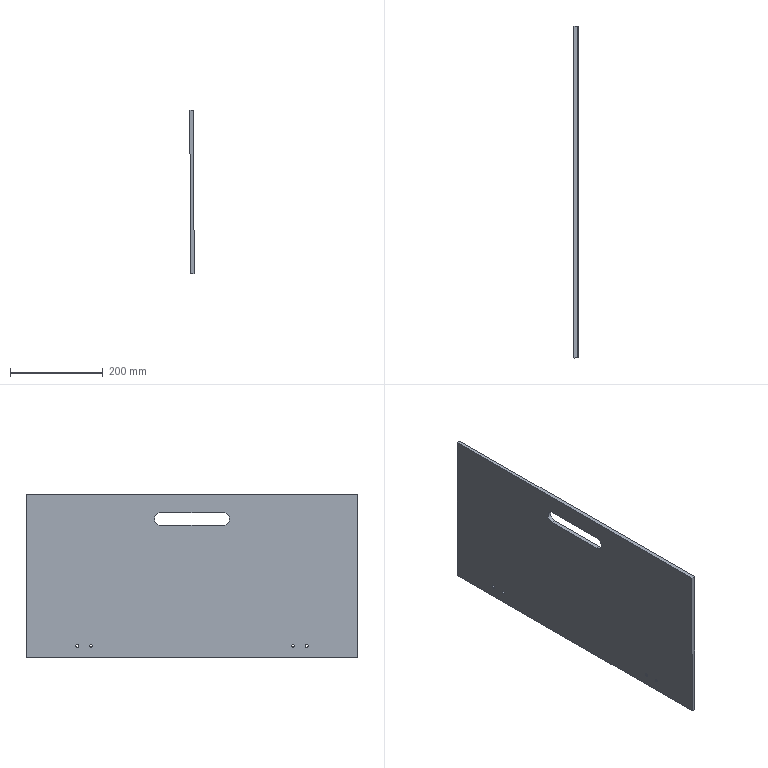Component | SolidWorks | FrameAssembly-1_LeftGlassDoor-1 | 1 solid | 18 faces | box 9.35 x 716 x 352.03 mm | volume 1981611 mm3 | cylinder 10 | plane 8 | commonest cylinder face diameters 6 x8 27 x2
build123d program:
from build123d import *

# Parameters (mm, degrees)
SKETCH1_W           = 352
SKETCH1_H           = 716
SKETCH1_R           = 3
BOSS_EXTRUDE1_DEPTH = 8


with BuildPart() as part:
    # Sketch1 → Boss-Extrude1 (new body)
    with BuildSketch(Plane.XY.offset(8)):
        Rectangle(SKETCH1_W, SKETCH1_H)
        with Locations(Location((-151, -218, 0), (0, 0, 180))):
            Circle(SKETCH1_R, mode=Mode.SUBTRACT)
        with Locations(Location((-151, 218, 0), (0, 0, 180))):
            Circle(SKETCH1_R, mode=Mode.SUBTRACT)
        with Locations(Location((-151, 248, 0), (0, 0, 180))):
            Circle(SKETCH1_R, mode=Mode.SUBTRACT)
        with Locations(Location((-151, -248, 0), (0, 0, 180))):
            Circle(SKETCH1_R, mode=Mode.SUBTRACT)
        with BuildLine():
            Line((109.5, -67.5), (109.5, 67.5))
            ThreePointArc((109.5, 67.5), (123, 81), (136.5, 67.5))
            Line((136.5, 67.5), (136.5, -67.5))
            ThreePointArc((136.5, -67.5), (123, -81), (109.5, -67.5))
        make_face(mode=Mode.SUBTRACT)
    extrude(amount=-BOSS_EXTRUDE1_DEPTH)


solid = part.part

# Placed as in the assembly
solid = solid.moved(Location((-661.912, -38.627, 160.537), (0, 89.781, 180)))
STEP:
#1=COLOUR_RGB('',0.7922,0.8196,0.9333);
#2=FILL_AREA_STYLE_COLOUR('',#1);
#3=FILL_AREA_STYLE('',(#2));
#4=SURFACE_STYLE_FILL_AREA(#3);
#5=SURFACE_SIDE_STYLE('',(#4));
#6=SURFACE_STYLE_USAGE(.BOTH.,#5);
#7=PRESENTATION_STYLE_ASSIGNMENT((#6));
#8=CARTESIAN_POINT('',(-25.721,-11.285,0.2586));
#9=VERTEX_POINT('',#8);
#10=CARTESIAN_POINT('',(-25.722,-11.285,0.4948));
#11=VERTEX_POINT('',#10);
#12=CARTESIAN_POINT('',(-25.722,-11.285,0.3767));
#13=DIRECTION('',(-1.,0.,-0.003827));
#14=DIRECTION('',(0.003827,0.,-1.));
#15=AXIS2_PLACEMENT_3D('',#12,#13,#14);
#16=CIRCLE('',#15,0.1181);
#17=EDGE_CURVE('',#9,#11,#16,.T.);
#18=ORIENTED_EDGE('',*,*,#17,.F.);
#19=CARTESIAN_POINT('',(-26.036,-11.285,0.2574));
#20=VERTEX_POINT('',#19);
#21=CARTESIAN_POINT('',(-25.721,-11.285,0.2586));
#22=DIRECTION('',(-1.,0.,-0.003827));
#23=VECTOR('',#22,39.37);
#24=LINE('',#21,#23);
#25=EDGE_CURVE('',#9,#20,#24,.T.);
#26=ORIENTED_EDGE('',*,*,#25,.T.);
#27=CARTESIAN_POINT('',(-26.037,-11.285,0.4936));
#28=VERTEX_POINT('',#27);
#29=CARTESIAN_POINT('',(-26.037,-11.285,0.3755));
#30=DIRECTION('',(-1.,0.,-0.003827));
#31=DIRECTION('',(0.003827,0.,-1.));
#32=AXIS2_PLACEMENT_3D('',#29,#30,#31);
#33=CIRCLE('',#32,0.1181);
#34=EDGE_CURVE('',#20,#28,#33,.T.);
#35=ORIENTED_EDGE('',*,*,#34,.T.);
#36=CARTESIAN_POINT('',(-25.722,-11.285,0.4948));
#37=DIRECTION('',(-1.,0.,-0.003827));
#38=VECTOR('',#37,39.37);
#39=LINE('',#36,#38);
#40=EDGE_CURVE('',#11,#28,#39,.T.);
#41=ORIENTED_EDGE('',*,*,#40,.F.);
#42=EDGE_LOOP('',(#18,#26,#35,#41));
#43=FACE_OUTER_BOUND('',#42,.T.);
#44=CARTESIAN_POINT('',(-25.722,-11.285,0.3767));
#45=DIRECTION('',(-1.,0.,-0.003827));
#46=DIRECTION('',(-0.003827,0.,1.));
#47=AXIS2_PLACEMENT_3D('',#44,#45,#46);
#48=CYLINDRICAL_SURFACE('',#47,0.1181);
#49=ADVANCED_FACE('',(#43),#48,.F.);
#50=CARTESIAN_POINT('',(-25.721,8.243,0.2586));
#51=VERTEX_POINT('',#50);
#52=CARTESIAN_POINT('',(-25.722,8.243,0.4948));
#53=VERTEX_POINT('',#52);
#54=CARTESIAN_POINT('',(-25.722,8.243,0.3767));
#55=DIRECTION('',(-1.,0.,-0.003827));
#56=DIRECTION('',(0.003827,0.,-1.));
#57=AXIS2_PLACEMENT_3D('',#54,#55,#56);
#58=CIRCLE('',#57,0.1181);
#59=EDGE_CURVE('',#51,#53,#58,.T.);
#60=ORIENTED_EDGE('',*,*,#59,.F.);
#61=CARTESIAN_POINT('',(-26.036,8.243,0.2574));
#62=VERTEX_POINT('',#61);
#63=CARTESIAN_POINT('',(-25.721,8.243,0.2586));
#64=DIRECTION('',(-1.,0.,-0.003827));
#65=VECTOR('',#64,39.37);
#66=LINE('',#63,#65);
#67=EDGE_CURVE('',#51,#62,#66,.T.);
#68=ORIENTED_EDGE('',*,*,#67,.T.);
#69=CARTESIAN_POINT('',(-26.037,8.243,0.4936));
#70=VERTEX_POINT('',#69);
#71=CARTESIAN_POINT('',(-26.037,8.243,0.3755));
#72=DIRECTION('',(-1.,0.,-0.003827));
#73=DIRECTION('',(0.003827,0.,-1.));
#74=AXIS2_PLACEMENT_3D('',#71,#72,#73);
#75=CIRCLE('',#74,0.1181);
#76=EDGE_CURVE('',#62,#70,#75,.T.);
#77=ORIENTED_EDGE('',*,*,#76,.T.);
#78=CARTESIAN_POINT('',(-25.722,8.243,0.4948));
#79=DIRECTION('',(-1.,0.,-0.003827));
#80=VECTOR('',#79,39.37);
#81=LINE('',#78,#80);
#82=EDGE_CURVE('',#53,#70,#81,.T.);
#83=ORIENTED_EDGE('',*,*,#82,.F.);
#84=EDGE_LOOP('',(#60,#68,#77,#83));
#85=FACE_OUTER_BOUND('',#84,.T.);
#86=CARTESIAN_POINT('',(-25.722,8.243,0.3767));
#87=DIRECTION('',(-1.,0.,-0.003827));
#88=DIRECTION('',(-0.003827,0.,1.));
#89=AXIS2_PLACEMENT_3D('',#86,#87,#88);
#90=CYLINDRICAL_SURFACE('',#89,0.1181);
#91=ADVANCED_FACE('',(#85),#90,.F.);
#92=CARTESIAN_POINT('',(-25.721,7.062,0.2586));
#93=VERTEX_POINT('',#92);
#94=CARTESIAN_POINT('',(-25.722,7.062,0.4948));
#95=VERTEX_POINT('',#94);
#96=CARTESIAN_POINT('',(-25.722,7.062,0.3767));
#97=DIRECTION('',(-1.,0.,-0.003827));
#98=DIRECTION('',(0.003827,0.,-1.));
#99=AXIS2_PLACEMENT_3D('',#96,#97,#98);
#100=CIRCLE('',#99,0.1181);
#101=EDGE_CURVE('',#93,#95,#100,.T.);
#102=ORIENTED_EDGE('',*,*,#101,.F.);
#103=CARTESIAN_POINT('',(-26.036,7.062,0.2574));
#104=VERTEX_POINT('',#103);
#105=CARTESIAN_POINT('',(-25.721,7.062,0.2586));
#106=DIRECTION('',(-1.,0.,-0.003827));
#107=VECTOR('',#106,39.37);
#108=LINE('',#105,#107);
#109=EDGE_CURVE('',#93,#104,#108,.T.);
#110=ORIENTED_EDGE('',*,*,#109,.T.);
#111=CARTESIAN_POINT('',(-26.037,7.062,0.4936));
#112=VERTEX_POINT('',#111);
#113=CARTESIAN_POINT('',(-26.037,7.062,0.3755));
#114=DIRECTION('',(-1.,0.,-0.003827));
#115=DIRECTION('',(0.003827,0.,-1.));
#116=AXIS2_PLACEMENT_3D('',#113,#114,#115);
#117=CIRCLE('',#116,0.1181);
#118=EDGE_CURVE('',#104,#112,#117,.T.);
#119=ORIENTED_EDGE('',*,*,#118,.T.);
#120=CARTESIAN_POINT('',(-25.722,7.062,0.4948));
#121=DIRECTION('',(-1.,0.,-0.003827));
#122=VECTOR('',#121,39.37);
#123=LINE('',#120,#122);
#124=EDGE_CURVE('',#95,#112,#123,.T.);
#125=ORIENTED_EDGE('',*,*,#124,.F.);
#126=EDGE_LOOP('',(#102,#110,#119,#125));
#127=FACE_OUTER_BOUND('',#126,.T.);
#128=CARTESIAN_POINT('',(-25.722,7.062,0.3767));
#129=DIRECTION('',(-1.,0.,-0.003827));
#130=DIRECTION('',(-0.003827,0.,1.));
#131=AXIS2_PLACEMENT_3D('',#128,#129,#130);
#132=CYLINDRICAL_SURFACE('',#131,0.1181);
#133=ADVANCED_FACE('',(#127),#132,.F.);
#134=CARTESIAN_POINT('',(-25.721,-10.103,0.2586));
#135=VERTEX_POINT('',#134);
#136=CARTESIAN_POINT('',(-25.722,-10.103,0.4948));
#137=VERTEX_POINT('',#136);
#138=CARTESIAN_POINT('',(-25.722,-10.103,0.3767));
#139=DIRECTION('',(-1.,0.,-0.003827));
#140=DIRECTION('',(0.003827,0.,-1.));
#141=AXIS2_PLACEMENT_3D('',#138,#139,#140);
#142=CIRCLE('',#141,0.1181);
#143=EDGE_CURVE('',#135,#137,#142,.T.);
#144=ORIENTED_EDGE('',*,*,#143,.F.);
#145=CARTESIAN_POINT('',(-26.036,-10.103,0.2574));
#146=VERTEX_POINT('',#145);
#147=CARTESIAN_POINT('',(-25.721,-10.103,0.2586));
#148=DIRECTION('',(-1.,0.,-0.003827));
#149=VECTOR('',#148,39.37);
#150=LINE('',#147,#149);
#151=EDGE_CURVE('',#135,#146,#150,.T.);
#152=ORIENTED_EDGE('',*,*,#151,.T.);
#153=CARTESIAN_POINT('',(-26.037,-10.103,0.4936));
#154=VERTEX_POINT('',#153);
#155=CARTESIAN_POINT('',(-26.037,-10.103,0.3755));
#156=DIRECTION('',(-1.,0.,-0.003827));
#157=DIRECTION('',(0.003827,0.,-1.));
#158=AXIS2_PLACEMENT_3D('',#155,#156,#157);
#159=CIRCLE('',#158,0.1181);
#160=EDGE_CURVE('',#146,#154,#159,.T.);
#161=ORIENTED_EDGE('',*,*,#160,.T.);
#162=CARTESIAN_POINT('',(-25.722,-10.103,0.4948));
#163=DIRECTION('',(-1.,0.,-0.003827));
#164=VECTOR('',#163,39.37);
#165=LINE('',#162,#164);
#166=EDGE_CURVE('',#137,#154,#165,.T.);
#167=ORIENTED_EDGE('',*,*,#166,.F.);
#168=EDGE_LOOP('',(#144,#152,#161,#167));
#169=FACE_OUTER_BOUND('',#168,.T.);
#170=CARTESIAN_POINT('',(-25.722,-10.103,0.3767));
#171=DIRECTION('',(-1.,0.,-0.003827));
#172=DIRECTION('',(-0.003827,0.,1.));
#173=AXIS2_PLACEMENT_3D('',#170,#171,#172);
#174=CYLINDRICAL_SURFACE('',#173,0.1181);
#175=ADVANCED_FACE('',(#169),#174,.F.);
#176=CARTESIAN_POINT('',(-26.086,12.574,13.249));
#177=VERTEX_POINT('',#176);
#178=CARTESIAN_POINT('',(-26.033,12.574,-0.6087));
#179=VERTEX_POINT('',#178);
#180=CARTESIAN_POINT('',(-26.086,12.574,13.249));
#181=DIRECTION('',(0.003827,-0.,-1.));
#182=VECTOR('',#181,39.37);
#183=LINE('',#180,#182);
#184=EDGE_CURVE('',#177,#179,#183,.T.);
#185=ORIENTED_EDGE('',*,*,#184,.F.);
#186=CARTESIAN_POINT('',(-25.771,12.574,13.251));
#187=VERTEX_POINT('',#186);
#188=CARTESIAN_POINT('',(-25.771,12.574,13.251));
#189=DIRECTION('',(-1.,0.,-0.003827));
#190=VECTOR('',#189,39.37);
#191=LINE('',#188,#190);
#192=EDGE_CURVE('',#187,#177,#191,.T.);
#193=ORIENTED_EDGE('',*,*,#192,.F.);
#194=CARTESIAN_POINT('',(-25.718,12.574,-0.6075));
#195=VERTEX_POINT('',#194);
#196=CARTESIAN_POINT('',(-25.771,12.574,13.251));
#197=DIRECTION('',(0.003827,-0.,-1.));
#198=VECTOR('',#197,39.37);
#199=LINE('',#196,#198);
#200=EDGE_CURVE('',#187,#195,#199,.T.);
#201=ORIENTED_EDGE('',*,*,#200,.T.);
#202=CARTESIAN_POINT('',(-25.718,12.574,-0.6075));
#203=DIRECTION('',(-1.,0.,-0.003827));
#204=VECTOR('',#203,39.37);
#205=LINE('',#202,#204);
#206=EDGE_CURVE('',#195,#179,#205,.T.);
#207=ORIENTED_EDGE('',*,*,#206,.T.);
#208=EDGE_LOOP('',(#185,#193,#201,#207));
#209=FACE_OUTER_BOUND('',#208,.T.);
#210=CARTESIAN_POINT('',(-25.771,12.574,13.251));
#211=DIRECTION('',(0.,1.,-0.));
#212=DIRECTION('',(-1.,0.,-0.003827));
#213=AXIS2_PLACEMENT_3D('',#210,#211,#212);
#214=PLANE('',#213);
#215=ADVANCED_FACE('',(#209),#214,.T.);
#216=CARTESIAN_POINT('',(-26.086,-15.615,13.249));
#217=VERTEX_POINT('',#216);
#218=CARTESIAN_POINT('',(-26.086,-15.615,13.249));
#219=DIRECTION('',(0.,1.,-0.));
#220=VECTOR('',#219,39.37);
#221=LINE('',#218,#220);
#222=EDGE_CURVE('',#217,#177,#221,.T.);
#223=ORIENTED_EDGE('',*,*,#222,.F.);
#224=CARTESIAN_POINT('',(-25.771,-15.615,13.251));
#225=VERTEX_POINT('',#224);
#226=CARTESIAN_POINT('',(-25.771,-15.615,13.251));
#227=DIRECTION('',(-1.,0.,-0.003827));
#228=VECTOR('',#227,39.37);
#229=LINE('',#226,#228);
#230=EDGE_CURVE('',#225,#217,#229,.T.);
#231=ORIENTED_EDGE('',*,*,#230,.F.);
#232=CARTESIAN_POINT('',(-25.771,-15.615,13.251));
#233=DIRECTION('',(0.,1.,-0.));
#234=VECTOR('',#233,39.37);
#235=LINE('',#232,#234);
#236=EDGE_CURVE('',#225,#187,#235,.T.);
#237=ORIENTED_EDGE('',*,*,#236,.T.);
#238=ORIENTED_EDGE('',*,*,#192,.T.);
#239=EDGE_LOOP('',(#223,#231,#237,#238));
#240=FACE_OUTER_BOUND('',#239,.T.);
#241=CARTESIAN_POINT('',(-25.771,-15.615,13.251));
#242=DIRECTION('',(-0.003827,0.,1.));
#243=DIRECTION('',(1.,-0.,0.003827));
#244=AXIS2_PLACEMENT_3D('',#241,#242,#243);
#245=PLANE('',#244);
#246=ADVANCED_FACE('',(#240),#245,.T.);
#247=CARTESIAN_POINT('',(-26.033,-15.615,-0.6087));
#248=VERTEX_POINT('',#247);
#249=CARTESIAN_POINT('',(-26.033,-15.615,-0.6087));
#250=DIRECTION('',(-0.003827,0.,1.));
#251=VECTOR('',#250,39.37);
#252=LINE('',#249,#251);
#253=EDGE_CURVE('',#248,#217,#252,.T.);
#254=ORIENTED_EDGE('',*,*,#253,.F.);
#255=CARTESIAN_POINT('',(-25.718,-15.615,-0.6075));
#256=VERTEX_POINT('',#255);
#257=CARTESIAN_POINT('',(-25.718,-15.615,-0.6075));
#258=DIRECTION('',(-1.,0.,-0.003827));
#259=VECTOR('',#258,39.37);
#260=LINE('',#257,#259);
#261=EDGE_CURVE('',#256,#248,#260,.T.);
#262=ORIENTED_EDGE('',*,*,#261,.F.);
#263=CARTESIAN_POINT('',(-25.718,-15.615,-0.6075));
#264=DIRECTION('',(-0.003827,0.,1.));
#265=VECTOR('',#264,39.37);
#266=LINE('',#263,#265);
#267=EDGE_CURVE('',#256,#225,#266,.T.);
#268=ORIENTED_EDGE('',*,*,#267,.T.);
#269=ORIENTED_EDGE('',*,*,#230,.T.);
#270=EDGE_LOOP('',(#254,#262,#268,#269));
#271=FACE_OUTER_BOUND('',#270,.T.);
#272=CARTESIAN_POINT('',(-25.718,-15.615,-0.6075));
#273=DIRECTION('',(-0.,-1.,0.));
#274=DIRECTION('',(1.,-0.,0.003827));
#275=AXIS2_PLACEMENT_3D('',#272,#273,#274);
#276=PLANE('',#275);
#277=ADVANCED_FACE('',(#271),#276,.T.);
#278=CARTESIAN_POINT('',(-26.033,12.574,-0.6087));
#279=DIRECTION('',(-0.,-1.,0.));
#280=VECTOR('',#279,39.37);
#281=LINE('',#278,#280);
#282=EDGE_CURVE('',#179,#248,#281,.T.);
#283=ORIENTED_EDGE('',*,*,#282,.F.);
#284=ORIENTED_EDGE('',*,*,#206,.F.);
#285=CARTESIAN_POINT('',(-25.718,12.574,-0.6075));
#286=DIRECTION('',(-0.,-1.,0.));
#287=VECTOR('',#286,39.37);
#288=LINE('',#285,#287);
#289=EDGE_CURVE('',#195,#256,#288,.T.);
#290=ORIENTED_EDGE('',*,*,#289,.T.);
#291=ORIENTED_EDGE('',*,*,#261,.T.);
#292=EDGE_LOOP('',(#283,#284,#290,#291));
#293=FACE_OUTER_BOUND('',#292,.T.);
#294=CARTESIAN_POINT('',(-25.718,12.574,-0.6075));
#295=DIRECTION('',(0.003827,-0.,-1.));
#296=DIRECTION('',(-1.,0.,-0.003827));
#297=AXIS2_PLACEMENT_3D('',#294,#295,#296);
#298=PLANE('',#297);
#299=ADVANCED_FACE('',(#293),#298,.T.);
#300=CARTESIAN_POINT('',(-25.722,-11.285,0.3767));
#301=DIRECTION('',(-1.,0.,-0.003827));
#302=DIRECTION('',(0.003827,0.,-1.));
#303=AXIS2_PLACEMENT_3D('',#300,#301,#302);
#304=CIRCLE('',#303,0.1181);
#305=EDGE_CURVE('',#11,#9,#304,.T.);
#306=ORIENTED_EDGE('',*,*,#305,.T.);
#307=ORIENTED_EDGE('',*,*,#17,.T.);
#308=EDGE_LOOP('',(#306,#307));
#309=FACE_BOUND('',#308,.T.);
#310=CARTESIAN_POINT('',(-25.761,1.137,10.633));
#311=VERTEX_POINT('',#310);
#312=CARTESIAN_POINT('',(-25.761,-4.178,10.633));
#313=VERTEX_POINT('',#312);
#314=CARTESIAN_POINT('',(-25.761,-4.178,10.633));
#315=DIRECTION('',(-0.,-1.,0.));
#316=VECTOR('',#315,39.37);
#317=LINE('',#314,#316);
#318=EDGE_CURVE('',#311,#313,#317,.T.);
#319=ORIENTED_EDGE('',*,*,#318,.T.);
#320=CARTESIAN_POINT('',(-25.765,-4.178,11.696));
#321=VERTEX_POINT('',#320);
#322=CARTESIAN_POINT('',(-25.763,-4.178,11.164));
#323=DIRECTION('',(-1.,0.,-0.003827));
#324=DIRECTION('',(0.003827,0.,-1.));
#325=AXIS2_PLACEMENT_3D('',#322,#323,#324);
#326=CIRCLE('',#325,0.5315);
#327=EDGE_CURVE('',#313,#321,#326,.T.);
#328=ORIENTED_EDGE('',*,*,#327,.T.);
#329=CARTESIAN_POINT('',(-25.765,1.137,11.696));
#330=VERTEX_POINT('',#329);
#331=CARTESIAN_POINT('',(-25.765,1.137,11.696));
#332=DIRECTION('',(0.,1.,-0.));
#333=VECTOR('',#332,39.37);
#334=LINE('',#331,#333);
#335=EDGE_CURVE('',#321,#330,#334,.T.);
#336=ORIENTED_EDGE('',*,*,#335,.T.);
#337=CARTESIAN_POINT('',(-25.763,1.137,11.164));
#338=DIRECTION('',(-1.,0.,-0.003827));
#339=DIRECTION('',(0.003827,0.,-1.));
#340=AXIS2_PLACEMENT_3D('',#337,#338,#339);
#341=CIRCLE('',#340,0.5315);
#342=EDGE_CURVE('',#330,#311,#341,.T.);
#343=ORIENTED_EDGE('',*,*,#342,.T.);
#344=EDGE_LOOP('',(#319,#328,#336,#343));
#345=FACE_BOUND('',#344,.T.);
#346=CARTESIAN_POINT('',(-25.722,8.243,0.3767));
#347=DIRECTION('',(-1.,0.,-0.003827));
#348=DIRECTION('',(0.003827,0.,-1.));
#349=AXIS2_PLACEMENT_3D('',#346,#347,#348);
#350=CIRCLE('',#349,0.1181);
#351=EDGE_CURVE('',#53,#51,#350,.T.);
#352=ORIENTED_EDGE('',*,*,#351,.T.);
#353=ORIENTED_EDGE('',*,*,#59,.T.);
#354=EDGE_LOOP('',(#352,#353));
#355=FACE_BOUND('',#354,.T.);
#356=CARTESIAN_POINT('',(-25.722,7.062,0.3767));
#357=DIRECTION('',(-1.,0.,-0.003827));
#358=DIRECTION('',(0.003827,0.,-1.));
#359=AXIS2_PLACEMENT_3D('',#356,#357,#358);
#360=CIRCLE('',#359,0.1181);
#361=EDGE_CURVE('',#95,#93,#360,.T.);
#362=ORIENTED_EDGE('',*,*,#361,.T.);
#363=ORIENTED_EDGE('',*,*,#101,.T.);
#364=EDGE_LOOP('',(#362,#363));
#365=FACE_BOUND('',#364,.T.);
#366=CARTESIAN_POINT('',(-25.722,-10.103,0.3767));
#367=DIRECTION('',(-1.,0.,-0.003827));
#368=DIRECTION('',(0.003827,0.,-1.));
#369=AXIS2_PLACEMENT_3D('',#366,#367,#368);
#370=CIRCLE('',#369,0.1181);
#371=EDGE_CURVE('',#137,#135,#370,.T.);
#372=ORIENTED_EDGE('',*,*,#371,.T.);
#373=ORIENTED_EDGE('',*,*,#143,.T.);
#374=EDGE_LOOP('',(#372,#373));
#375=FACE_BOUND('',#374,.T.);
#376=ORIENTED_EDGE('',*,*,#200,.F.);
#377=ORIENTED_EDGE('',*,*,#236,.F.);
#378=ORIENTED_EDGE('',*,*,#267,.F.);
#379=ORIENTED_EDGE('',*,*,#289,.F.);
#380=EDGE_LOOP('',(#376,#377,#378,#379));
#381=FACE_OUTER_BOUND('',#380,.T.);
#382=CARTESIAN_POINT('',(-25.745,-1.521,6.322));
#383=DIRECTION('',(-1.,0.,-0.003827));
#384=DIRECTION('',(-0.003827,0.,1.));
#385=AXIS2_PLACEMENT_3D('',#382,#383,#384);
#386=PLANE('',#385);
#387=ADVANCED_FACE('',(#309,#345,#355,#365,#375,#381),#386,.F.);
#388=CARTESIAN_POINT('',(-26.037,-11.285,0.3755));
#389=DIRECTION('',(-1.,0.,-0.003827));
#390=DIRECTION('',(0.003827,0.,-1.));
#391=AXIS2_PLACEMENT_3D('',#388,#389,#390);
#392=CIRCLE('',#391,0.1181);
#393=EDGE_CURVE('',#28,#20,#392,.T.);
#394=ORIENTED_EDGE('',*,*,#393,.F.);
#395=ORIENTED_EDGE('',*,*,#34,.F.);
#396=EDGE_LOOP('',(#394,#395));
#397=FACE_BOUND('',#396,.T.);
#398=CARTESIAN_POINT('',(-26.076,-4.178,10.631));
#399=VERTEX_POINT('',#398);
#400=CARTESIAN_POINT('',(-26.08,-4.178,11.694));
#401=VERTEX_POINT('',#400);
#402=CARTESIAN_POINT('',(-26.078,-4.178,11.163));
#403=DIRECTION('',(-1.,0.,-0.003827));
#404=DIRECTION('',(0.003827,0.,-1.));
#405=AXIS2_PLACEMENT_3D('',#402,#403,#404);
#406=CIRCLE('',#405,0.5315);
#407=EDGE_CURVE('',#399,#401,#406,.T.);
#408=ORIENTED_EDGE('',*,*,#407,.F.);
#409=CARTESIAN_POINT('',(-26.076,1.137,10.631));
#410=VERTEX_POINT('',#409);
#411=CARTESIAN_POINT('',(-26.076,-4.178,10.631));
#412=DIRECTION('',(-0.,-1.,0.));
#413=VECTOR('',#412,39.37);
#414=LINE('',#411,#413);
#415=EDGE_CURVE('',#410,#399,#414,.T.);
#416=ORIENTED_EDGE('',*,*,#415,.F.);
#417=CARTESIAN_POINT('',(-26.08,1.137,11.694));
#418=VERTEX_POINT('',#417);
#419=CARTESIAN_POINT('',(-26.078,1.137,11.163));
#420=DIRECTION('',(-1.,0.,-0.003827));
#421=DIRECTION('',(0.003827,0.,-1.));
#422=AXIS2_PLACEMENT_3D('',#419,#420,#421);
#423=CIRCLE('',#422,0.5315);
#424=EDGE_CURVE('',#418,#410,#423,.T.);
#425=ORIENTED_EDGE('',*,*,#424,.F.);
#426=CARTESIAN_POINT('',(-26.08,1.137,11.694));
#427=DIRECTION('',(0.,1.,-0.));
#428=VECTOR('',#427,39.37);
#429=LINE('',#426,#428);
#430=EDGE_CURVE('',#401,#418,#429,.T.);
#431=ORIENTED_EDGE('',*,*,#430,.F.);
#432=EDGE_LOOP('',(#408,#416,#425,#431));
#433=FACE_BOUND('',#432,.T.);
#434=CARTESIAN_POINT('',(-26.037,8.243,0.3755));
#435=DIRECTION('',(-1.,0.,-0.003827));
#436=DIRECTION('',(0.003827,0.,-1.));
#437=AXIS2_PLACEMENT_3D('',#434,#435,#436);
#438=CIRCLE('',#437,0.1181);
#439=EDGE_CURVE('',#70,#62,#438,.T.);
#440=ORIENTED_EDGE('',*,*,#439,.F.);
#441=ORIENTED_EDGE('',*,*,#76,.F.);
#442=EDGE_LOOP('',(#440,#441));
#443=FACE_BOUND('',#442,.T.);
#444=CARTESIAN_POINT('',(-26.037,7.062,0.3755));
#445=DIRECTION('',(-1.,0.,-0.003827));
#446=DIRECTION('',(0.003827,0.,-1.));
#447=AXIS2_PLACEMENT_3D('',#444,#445,#446);
#448=CIRCLE('',#447,0.1181);
#449=EDGE_CURVE('',#112,#104,#448,.T.);
#450=ORIENTED_EDGE('',*,*,#449,.F.);
#451=ORIENTED_EDGE('',*,*,#118,.F.);
#452=EDGE_LOOP('',(#450,#451));
#453=FACE_BOUND('',#452,.T.);
#454=CARTESIAN_POINT('',(-26.037,-10.103,0.3755));
#455=DIRECTION('',(-1.,0.,-0.003827));
#456=DIRECTION('',(0.003827,0.,-1.));
#457=AXIS2_PLACEMENT_3D('',#454,#455,#456);
#458=CIRCLE('',#457,0.1181);
#459=EDGE_CURVE('',#154,#146,#458,.T.);
#460=ORIENTED_EDGE('',*,*,#459,.F.);
#461=ORIENTED_EDGE('',*,*,#160,.F.);
#462=EDGE_LOOP('',(#460,#461));
#463=FACE_BOUND('',#462,.T.);
#464=ORIENTED_EDGE('',*,*,#184,.T.);
#465=ORIENTED_EDGE('',*,*,#282,.T.);
#466=ORIENTED_EDGE('',*,*,#253,.T.);
#467=ORIENTED_EDGE('',*,*,#222,.T.);
#468=EDGE_LOOP('',(#464,#465,#466,#467));
#469=FACE_OUTER_BOUND('',#468,.T.);
#470=CARTESIAN_POINT('',(-26.06,-1.521,6.32));
#471=DIRECTION('',(-1.,0.,-0.003827));
#472=DIRECTION('',(-0.003827,0.,1.));
#473=AXIS2_PLACEMENT_3D('',#470,#471,#472);
#474=PLANE('',#473);
#475=ADVANCED_FACE('',(#397,#433,#443,#453,#463,#469),#474,.T.);
#476=ORIENTED_EDGE('',*,*,#151,.F.);
#477=ORIENTED_EDGE('',*,*,#371,.F.);
#478=ORIENTED_EDGE('',*,*,#166,.T.);
#479=ORIENTED_EDGE('',*,*,#459,.T.);
#480=EDGE_LOOP('',(#476,#477,#478,#479));
#481=FACE_OUTER_BOUND('',#480,.T.);
#482=CARTESIAN_POINT('',(-25.722,-10.103,0.3767));
#483=DIRECTION('',(-1.,0.,-0.003827));
#484=DIRECTION('',(-0.003827,0.,1.));
#485=AXIS2_PLACEMENT_3D('',#482,#483,#484);
#486=CYLINDRICAL_SURFACE('',#485,0.1181);
#487=ADVANCED_FACE('',(#481),#486,.F.);
#488=ORIENTED_EDGE('',*,*,#109,.F.);
#489=ORIENTED_EDGE('',*,*,#361,.F.);
#490=ORIENTED_EDGE('',*,*,#124,.T.);
#491=ORIENTED_EDGE('',*,*,#449,.T.);
#492=EDGE_LOOP('',(#488,#489,#490,#491));
#493=FACE_OUTER_BOUND('',#492,.T.);
#494=CARTESIAN_POINT('',(-25.722,7.062,0.3767));
#495=DIRECTION('',(-1.,0.,-0.003827));
#496=DIRECTION('',(-0.003827,0.,1.));
#497=AXIS2_PLACEMENT_3D('',#494,#495,#496);
#498=CYLINDRICAL_SURFACE('',#497,0.1181);
#499=ADVANCED_FACE('',(#493),#498,.F.);
#500=ORIENTED_EDGE('',*,*,#67,.F.);
#501=ORIENTED_EDGE('',*,*,#351,.F.);
#502=ORIENTED_EDGE('',*,*,#82,.T.);
#503=ORIENTED_EDGE('',*,*,#439,.T.);
#504=EDGE_LOOP('',(#500,#501,#502,#503));
#505=FACE_OUTER_BOUND('',#504,.T.);
#506=CARTESIAN_POINT('',(-25.722,8.243,0.3767));
#507=DIRECTION('',(-1.,0.,-0.003827));
#508=DIRECTION('',(-0.003827,0.,1.));
#509=AXIS2_PLACEMENT_3D('',#506,#507,#508);
#510=CYLINDRICAL_SURFACE('',#509,0.1181);
#511=ADVANCED_FACE('',(#505),#510,.F.);
#512=ORIENTED_EDGE('',*,*,#407,.T.);
#513=CARTESIAN_POINT('',(-25.765,-4.178,11.696));
#514=DIRECTION('',(-1.,0.,-0.003827));
#515=VECTOR('',#514,39.37);
#516=LINE('',#513,#515);
#517=EDGE_CURVE('',#321,#401,#516,.T.);
#518=ORIENTED_EDGE('',*,*,#517,.F.);
#519=ORIENTED_EDGE('',*,*,#327,.F.);
#520=CARTESIAN_POINT('',(-25.761,-4.178,10.633));
#521=DIRECTION('',(-1.,0.,-0.003827));
#522=VECTOR('',#521,39.37);
#523=LINE('',#520,#522);
#524=EDGE_CURVE('',#313,#399,#523,.T.);
#525=ORIENTED_EDGE('',*,*,#524,.T.);
#526=EDGE_LOOP('',(#512,#518,#519,#525));
#527=FACE_OUTER_BOUND('',#526,.T.);
#528=CARTESIAN_POINT('',(-25.763,-4.178,11.164));
#529=DIRECTION('',(-1.,0.,-0.003827));
#530=DIRECTION('',(-0.003827,0.,1.));
#531=AXIS2_PLACEMENT_3D('',#528,#529,#530);
#532=CYLINDRICAL_SURFACE('',#531,0.5315);
#533=ADVANCED_FACE('',(#527),#532,.F.);
#534=ORIENTED_EDGE('',*,*,#415,.T.);
#535=ORIENTED_EDGE('',*,*,#524,.F.);
#536=ORIENTED_EDGE('',*,*,#318,.F.);
#537=CARTESIAN_POINT('',(-25.761,1.137,10.633));
#538=DIRECTION('',(-1.,0.,-0.003827));
#539=VECTOR('',#538,39.37);
#540=LINE('',#537,#539);
#541=EDGE_CURVE('',#311,#410,#540,.T.);
#542=ORIENTED_EDGE('',*,*,#541,.T.);
#543=EDGE_LOOP('',(#534,#535,#536,#542));
#544=FACE_OUTER_BOUND('',#543,.T.);
#545=CARTESIAN_POINT('',(-25.761,-4.178,10.633));
#546=DIRECTION('',(0.003827,-0.,-1.));
#547=DIRECTION('',(-1.,0.,-0.003827));
#548=AXIS2_PLACEMENT_3D('',#545,#546,#547);
#549=PLANE('',#548);
#550=ADVANCED_FACE('',(#544),#549,.F.);
#551=ORIENTED_EDGE('',*,*,#424,.T.);
#552=ORIENTED_EDGE('',*,*,#541,.F.);
#553=ORIENTED_EDGE('',*,*,#342,.F.);
#554=CARTESIAN_POINT('',(-25.765,1.137,11.696));
#555=DIRECTION('',(-1.,0.,-0.003827));
#556=VECTOR('',#555,39.37);
#557=LINE('',#554,#556);
#558=EDGE_CURVE('',#330,#418,#557,.T.);
#559=ORIENTED_EDGE('',*,*,#558,.T.);
#560=EDGE_LOOP('',(#551,#552,#553,#559));
#561=FACE_OUTER_BOUND('',#560,.T.);
#562=CARTESIAN_POINT('',(-25.763,1.137,11.164));
#563=DIRECTION('',(-1.,0.,-0.003827));
#564=DIRECTION('',(-0.003827,0.,1.));
#565=AXIS2_PLACEMENT_3D('',#562,#563,#564);
#566=CYLINDRICAL_SURFACE('',#565,0.5315);
#567=ADVANCED_FACE('',(#561),#566,.F.);
#568=ORIENTED_EDGE('',*,*,#430,.T.);
#569=ORIENTED_EDGE('',*,*,#558,.F.);
#570=ORIENTED_EDGE('',*,*,#335,.F.);
#571=ORIENTED_EDGE('',*,*,#517,.T.);
#572=EDGE_LOOP('',(#568,#569,#570,#571));
#573=FACE_OUTER_BOUND('',#572,.T.);
#574=CARTESIAN_POINT('',(-25.765,1.137,11.696));
#575=DIRECTION('',(-0.003827,0.,1.));
#576=DIRECTION('',(1.,-0.,0.003827));
#577=AXIS2_PLACEMENT_3D('',#574,#575,#576);
#578=PLANE('',#577);
#579=ADVANCED_FACE('',(#573),#578,.F.);
#580=ORIENTED_EDGE('',*,*,#25,.F.);
#581=ORIENTED_EDGE('',*,*,#305,.F.);
#582=ORIENTED_EDGE('',*,*,#40,.T.);
#583=ORIENTED_EDGE('',*,*,#393,.T.);
#584=EDGE_LOOP('',(#580,#581,#582,#583));
#585=FACE_OUTER_BOUND('',#584,.T.);
#586=CARTESIAN_POINT('',(-25.722,-11.285,0.3767));
#587=DIRECTION('',(-1.,0.,-0.003827));
#588=DIRECTION('',(-0.003827,0.,1.));
#589=AXIS2_PLACEMENT_3D('',#586,#587,#588);
#590=CYLINDRICAL_SURFACE('',#589,0.1181);
#591=ADVANCED_FACE('',(#585),#590,.F.);
#592=CLOSED_SHELL('',(#49,#91,#133,#175,#215,#246,#277,#299,#387,#475,#487,#499,#511,#533,#550,#567,#579,#591));
#593=MANIFOLD_SOLID_BREP('',#592);
#594=STYLED_ITEM('',(#7),#593);
#595=PRESENTATION_LAYER_ASSIGNMENT('','',(#594));
#596=CARTESIAN_POINT('',(0.,0.,0.));
#597=DIRECTION('',(0.,0.,1.));
#598=DIRECTION('',(1.,0.,0.));
#599=AXIS2_PLACEMENT_3D('',#596,#597,#598);
#600=(LENGTH_UNIT()NAMED_UNIT(*)SI_UNIT($,.METRE.));
#601=LENGTH_MEASURE_WITH_UNIT(LENGTH_MEASURE(0.0254),#600);
#602=DIMENSIONAL_EXPONENTS(1.,0.,0.,0.,0.,0.,0.);
#603=(CONVERSION_BASED_UNIT('',#601)LENGTH_UNIT()NAMED_UNIT(#602));
#604=UNCERTAINTY_MEASURE_WITH_UNIT(LENGTH_MEASURE(0.00001),#603,'','');
#605=(NAMED_UNIT(*)PLANE_ANGLE_UNIT()SI_UNIT($,.RADIAN.));
#606=(NAMED_UNIT(*)SI_UNIT($,.STERADIAN.)SOLID_ANGLE_UNIT());
#607=(GEOMETRIC_REPRESENTATION_CONTEXT(3)GLOBAL_UNCERTAINTY_ASSIGNED_CONTEXT((#604))GLOBAL_UNIT_ASSIGNED_CONTEXT((#603,#605,#606))REPRESENTATION_CONTEXT('',''));
#608=ADVANCED_BREP_SHAPE_REPRESENTATION('',(#593,#599),#607);
#609=(LENGTH_UNIT()NAMED_UNIT(*)SI_UNIT($,.METRE.));
#610=LENGTH_MEASURE_WITH_UNIT(LENGTH_MEASURE(0.0254),#609);
#611=DIMENSIONAL_EXPONENTS(1.,0.,0.,0.,0.,0.,0.);
#612=(CONVERSION_BASED_UNIT('',#610)LENGTH_UNIT()NAMED_UNIT(#611));
#613=UNCERTAINTY_MEASURE_WITH_UNIT(LENGTH_MEASURE(0.00001),#612,'','');
#614=(NAMED_UNIT(*)PLANE_ANGLE_UNIT()SI_UNIT($,.RADIAN.));
#615=(NAMED_UNIT(*)SI_UNIT($,.STERADIAN.)SOLID_ANGLE_UNIT());
#616=(GEOMETRIC_REPRESENTATION_CONTEXT(3)GLOBAL_UNCERTAINTY_ASSIGNED_CONTEXT((#613))GLOBAL_UNIT_ASSIGNED_CONTEXT((#612,#614,#615))REPRESENTATION_CONTEXT('',''));
#617=MECHANICAL_DESIGN_GEOMETRIC_PRESENTATION_REPRESENTATION('',(#594),#616);